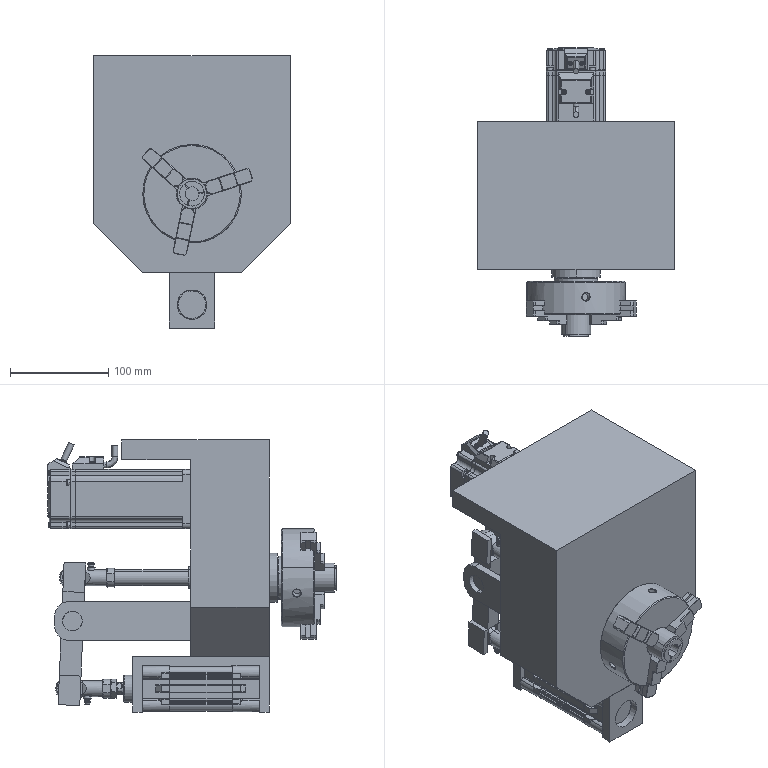Assembly | SolidWorks | mm | 28 component files | 28 solids | 2282 faces | box 200 x 292.9 x 276.5 mm | volume 4855471 mm3 | plane 1247 | cylinder 609 | cone 280 | spline 146 | commonest cylinder face diameters 1 x104 0.4 x44 8 x34 6 x32 5.5 x28 4 x25 5 x21 20 x20
Bill of materials:
HZ022-A001-D001 | 1 | AL6061 | Rectangular block with a thin flange running off one top edge, giving an L-shaped side profile. The front face has two chamfered lower corners and one round through hole, and a short cylindrical boss or sleeve sticks out slightly around the hole.
HZ022-A001-D003 | 1 | S45C | Plain straight round tube with a constant wall thickness and square-cut ends.
HZ022-A001-D004 | 1 | S45C | Long stepped cylindrical shaft with three diameters that get smaller toward one end. The opposite end is hollow, flares slightly outward, and is split lengthwise by three slots, like a collet.
HZ022-A001-D005 | 1 | AL6061 | U-shaped (bridge-shaped) bracket: a flat top plate with two parallel legs, each leg having one large round hole on a common axis.
HZ022-A001-D006 | 1 | AL6061 | Rectangular bar with one rounded end that is split by a slot into two parallel tines (a clevis or fork). A cross hole runs through both tines.
HZ022-A001-D007 | 1 | AL6061 | Link-like assembly of flat plates: a central rectangular plate with pairs of outer plates at both ends, joined by short cylindrical pins. A further cylindrical pin or boss crosses the middle of the central plate.
HZ022-F-M10X125U | 2 | AL6061 | Rod-end-style body: a round eye housing holding a ball-like inner ring with a bore, a cylindrical shank with a hollow end bore and a short collar, and a small nipple-shaped protrusion on the underside of the shank near the eye.
HZ022-SE32x25S (1) | 1 | AL6061 | Thin flat ring washer with six tabs spaced evenly around the outer edge, all bent up out of the ring plane at an angle.
HZ022-SE32x25S (10) | 1 | AL6061 | Stepped cylinder: a larger-diameter body with a hexagonal socket recess in one end, and a smaller coaxial pin with a chamfered tip coming out of the other end.
HZ022-SE32x25S (11) | 1 | AL6061 | Stepped cylinder: a larger-diameter body with a hexagonal socket recess in one end, and a smaller coaxial pin with a chamfered tip coming out of the other end.
HZ022-SE32x25S (12) | 1 | AL6061 | Stepped cylinder: a larger-diameter body with a hexagonal socket recess in one end, and a smaller coaxial pin with a chamfered tip coming out of the other end.
HZ022-SE32x25S (13) | 1 | AL6061 | Stepped turned body with a hexagonal socket in the top face. Below a thin top flange sits a rounded torus-like ring in a groove, then a larger cylindrical section with a chamfered lower edge, then a narrower tapered spigot.
HZ022-SE32x25S (14) | 1 | AL6061 | Rotationally symmetric plug-like part: a short cylindrical head with a hexagonal socket in the top, a thin top flange, a rounded ring sitting in a groove below the flange, a larger cylindrical body with chamfered lower edge, and a smaller tapered/stepped shank with a rounded end.
HZ022-SE32x25S (15) | 1 | AL6061 | Thin flat annular ring with six evenly spaced rectangular tabs on the outer edge, bent out of the ring plane at angles in side view.
HZ022-SE32x25S (2) | 1 | AL6061 | Elongated, roughly square-section body with four rounded corner lobes holding through-bores, a round cylindrical boss/rod end coming out of each end face, long slots along the side faces, and pairs of small round holes on the top face near each end.
HZ022-SE32x25S (3) | 1 | AL6061 | Long, slender, rotationally symmetric stepped shaft: an open tubular end with a bore, a group of four thin collar ribs near that end, a long narrower shank, and a small-diameter end pin after a short hexagonal or faceted step.
HZ022-SE32x25S (4) | 1 | AL6061 | Hexagonal nut-like block with a central plain round bore and chamfered corners on both faces.
HZ022-SE32x25S (5) | 1 | AL6061 | Solid stepped cylindrical pin: a larger-diameter cylindrical section with a shoulder that steps down to a longer smaller-diameter pin with a chamfered tip.
HZ022-SE32x25S (6) | 1 | AL6061 | Solid stepped cylindrical pin: a larger-diameter cylindrical section with a shoulder that steps down to a longer smaller-diameter pin with a chamfered tip.
HZ022-SE32x25S (7) | 1 | AL6061 | Solid stepped cylindrical pin: a larger-diameter cylindrical section with a shoulder that steps down to a longer smaller-diameter pin with a chamfered tip.
HZ022-SE32x25S (8) | 1 | AL6061 | Solid stepped cylindrical pin: a larger-diameter cylindrical section with a shoulder that steps down to a longer smaller-diameter pin with a chamfered tip.
HZ022-SE32x25S (9) | 1 | AL6061 | Stepped cylindrical pin with a larger cylindrical section that steps down to a longer smaller-diameter pin with a chamfered tip. The larger end has a hexagonal socket recess.
HZ022-Three-JawChuck | 1 |  | Thick disk with a central through-bore and a raised circular boss on one face. The opposite face has three radial T-shaped slots running from the bore to the rim, and there are small radial holes in the outer cylindrical surface.
HZ022-Three-JawChuckJaw | 3 |  | Stepped prismatic block with chamfered edges: a three-level staircase profile, a longitudinal groove along the top, two transverse grooves across the stepped face, and a finely serrated end face.
HZ022-X-Axis-MS-60ST-M01330-20P4(Servo400W) | 1 | 45 | Long body with a square cross-section and a square front flange that has four corner through-holes and rounded corners. A short raised circular boss sits on the flange face, and a cylindrical shaft with a keyway or flat sticks out from the centre. Two block-shaped housings sit on top of the body near the rear: one has a bent cylindrical lead coming out of it, and the angled rear housing has a straight cylindrical lead at an angle. Small round screw-head features are visible on the housings. The overall form looks like a flange-mounted rotary motor, but this is inferred from the shape only.
Mates:
1. coincident | HZ022-A001-D001-1 face at (-12.865, -71.602, 510) dir (0, 1, 0) | HZ022-X-Axis-MS-60ST-M01330-20P4(Servo400W)-1 face at (12.135, -71.602, 585) dir (0, -1, 0)
2. concentric | HZ022-A001-D001-1 face at (-12.865, -76.602, 560) dir (0, 1, 0) r 25 | HZ022-X-Axis-MS-60ST-M01330-20P4(Servo400W)-1 face at (-12.865, -74.602, 560) dir (0, 1, 0) r 25
3. parallel | HZ022-A001-D001-1 face at (87.135, -71.602, 600) dir (0, 0, -1) | HZ022-X-Axis-MS-60ST-M01330-20P4(Servo400W)-1 face at (17.135, 70.398, 590) dir (0, 0, 1)
4. coincident | HZ022-A001-D001-1 face at (-12.865, -159.602, 480) dir (0, -1, 0) | HZ022-Three-JawChuck-1 face at (-12.865, -159.602, 480) dir (0, 1, 0)
5. concentric | HZ022-A001-D001-1 face at (-12.865, -159.602, 480) dir (0, 1, 0) r 25 | HZ022-Three-JawChuck-1 face at (-12.865, -159.602, 480) dir (0, -1, 0) r 22
6. coincident | HZ022-Three-JawChuckJaw-1 face at (3.573, -183.602, 478.055) dir (0, 1, 0) | HZ022-Three-JawChuck-1 face at (49.8, -183.602, 508.057) dir (0, -1, 0)
7. coincident | HZ022-Three-JawChuckJaw-1 face at (3.573, -183.602, 478.055) dir (0.3135, 0, -0.9496) | HZ022-Three-JawChuck-1 face at (54.188, -188.602, 494.763) dir (-0.3135, 0, 0.9496)
8. distance | HZ022-Three-JawChuckJaw-1 face at (1.379, -183.602, 484.702) dir (-0.9496, 0, -0.3135) | HZ022-Three-JawChuck-1 axis at (-12.865, -196.602, 480) dir (0, 1, 0)
9. concentric | HZ022-Three-JawChuck-1 face at (-12.865, -197.602, 480) dir (0, 1, 0) r 15 | HZ022-A001-D003-1 face at (-12.865, -97.602, 480) dir (0, -1, 0) r 15
10. tangent | HZ022-Three-JawChuckJaw-1 face at (1.379, -183.602, 484.702) dir (-0.9496, 0, -0.3135) | HZ022-A001-D003-1 face at (-12.865, -97.602, 480) dir (0, -1, 0) r 15
11. distance | HZ022-A001-D003-1 face at (-12.865, -217.602, 480) dir (0, -1, 0) | HZ022-Three-JawChuck-1 face at (-12.865, -197.602, 480) dir (0, -1, 0)
12. concentric | HZ022-A001-D003-1 face at (-12.865, -217.602, 480) dir (0, 1, 0) r 12 | HZ022-A001-D004-1 face at (-12.865, -69.505, 480) dir (0, 1, 0) r 11
13. coincident | HZ022-A001-D001-1 face at (-12.865, -1.602, 400) dir (0, 0, -1) | HZ022-A001-D005-1 face at (-12.865, -82.102, 400) dir (0, 0, 1)
14. coincident | HZ022-A001-D001-1 face at (-12.865, -151.602, 510) dir (0, -1, 0) | HZ022-A001-D005-1 face at (-36.115, -151.602, 390) dir (0, -1, 0)
15. width | HZ022-A001-D005-1 face at (10.385, -12.602, 390) dir (1, 0, 0) | HZ022-A001-D005-1 face at (-36.115, -12.602, 390) dir (-1, 0, 0) | HZ022-A001-D001-1 face at (-112.865, -1.602, 510) dir (-1, 0, 0) | HZ022-A001-D001-1 face at (87.135, -1.602, 510) dir (1, 0, 0)
16. coincident | HZ022-SE32x25S-1/HZ022-SE32x25S (2)-1 face at (-12.865, -141.602, 367.25) dir (0, -1, 0) | HZ022-A001-D005-1 face at (10.385, -141.602, 343.5) dir (0, 1, 0)
17. coincident | HZ022-SE32x25S-1/HZ022-SE32x25S (2)-1 face at (-24.418, -50.102, 390) dir (0, 0, 1) | HZ022-A001-D005-1 face at (-12.865, -82.102, 390) dir (0, 0, -1)
18. width | HZ022-SE32x25S-1/HZ022-SE32x25S (2)-1 face at (-35.615, -50.102, 363.6) dir (-1, 0, 0) | HZ022-SE32x25S-1/HZ022-SE32x25S (2)-1 face at (9.885, -50.102, 370.9) dir (1, 0, 0) | HZ022-A001-D005-1 face at (10.385, -12.602, 390) dir (1, 0, 0) | HZ022-A001-D005-1 face at (-36.115, -12.602, 390) dir (-1, 0, 0)
19. concentric | HZ022-SE32x25S-1/HZ022-SE32x25S (3)-1 face at (-12.865, 14.014, 367.25) dir (0, -1, 0) r 5 | HZ022-F-M10X125U-1 face at (-12.865, 20.431, 367.25) dir (0, -1, 0) r 4.324
20. coincident | HZ022-SE32x25S-1/HZ022-SE32x25S (4)-1 face at (-8.845, 9.398, 368.628) dir (0, 1, 0) | HZ022-F-M10X125U-1 face at (-5.865, 9.398, 367.25) dir (0, -1, 0)
21. parallel | HZ022-A001-D005-1 face at (10.385, -12.602, 390) dir (1, 0, 0) | HZ022-F-M10X125U-1 face at (-5.865, 52.398, 363.536) dir (1, 0, 0)
22. concentric | HZ022-A001-D004-1 face at (-12.865, 5.495, 480) dir (0, 1, 0) r 5 | HZ022-F-M10X125U-2 face at (-12.865, 16.528, 480) dir (0, -1, 0) r 4.324
23. parallel | HZ022-A001-D001-1 face at (87.135, -1.602, 510) dir (1, 0, 0) | HZ022-F-M10X125U-2 face at (-5.865, 48.495, 483.714) dir (1, 0, 0)
24. coincident | HZ022-A001-D004-1 face at (-12.865, 5.495, 480) dir (0, 1, 0) | HZ022-F-M10X125U-2 face at (-19.865, 5.495, 480) dir (0, -1, 0)
25. coincident | HZ022-A001-D001-1 face at (-12.865, -71.602, 510) dir (0, 1, 0) | HZ022-A001-D006-1 face at (2.135, -71.602, 416) dir (0, -1, 0)
26. width | HZ022-A001-D006-1 face at (2.135, -2.602, 436) dir (1, 0, 0) | HZ022-A001-D006-1 face at (-27.865, -2.602, 436) dir (-1, 0, 0) | HZ022-A001-D001-1 face at (-112.865, -1.602, 510) dir (-1, 0, 0) | HZ022-A001-D001-1 face at (87.135, -1.602, 510) dir (1, 0, 0)
27. tangent | HZ022-F-M10X125U-1 face at (-12.865, 52.398, 367.25) dir (-1, 0, 0) r 5 | HZ022-A001-D007-1 face at (-19.865, 51.327, 365.561) dir (1, 0, 0) r 3
28. coincident | HZ022-F-M10X125U-1 face at (-5.865, 52.398, 363.536) dir (1, 0, 0) | HZ022-A001-D007-1 face at (-5.865, 48.938, 423.011) dir (-1, 0, 0)
29. tangent | HZ022-F-M10X125U-2 face at (-12.865, 48.495, 480) dir (1, 0, 0) r 5 | HZ022-A001-D007-1 face at (-19.865, 46.549, 480.462) dir (1, 0, 0) r 3
30. distance | HZ022-A001-D006-1 face at (2.135, 66.398, 416) dir (0, 0, -1) | HZ022-A001-D001-1 face at (-12.865, -1.602, 400) dir (0, 0, -1)
31. concentric | HZ022-A001-D006-1 face at (-27.865, 48.398, 436) dir (1, 0, 0) r 10 | HZ022-A001-D007-1 face at (-2.865, 48.398, 436) dir (-1, 0, 0) r 10
32. distance | HZ022-SE32x25S (4)-1 face at (-32, 4.02, 1.378) dir (-1, 0, 0) | HZ022-SE32x25S (3)-1 face at (-48, -2.061, -0.4807) dir (-1, 0, 0)
33. concentric | HZ022-SE32x25S (3)-1 face at (-36.617, 0, 0) dir (1, 0, 0) r 5 | HZ022-SE32x25S (4)-1 face at (-29, 0, 0) dir (1, 0, 0) r 4.324
34. concentric | HZ022-SE32x25S (2)-1 face at (-8.5, 0, 0) dir (1, 0, 0) r 6 | HZ022-SE32x25S (3)-1 face at (3.5, 0, 0) dir (1, 0, 0) r 6
35. distance | HZ022-SE32x25S (3)-1 face at (85, -11.467, -2.675) dir (1, 0, 0) | HZ022-SE32x25S (2)-1 face at (85, 12.025, 0) dir (-1, 0, 0)